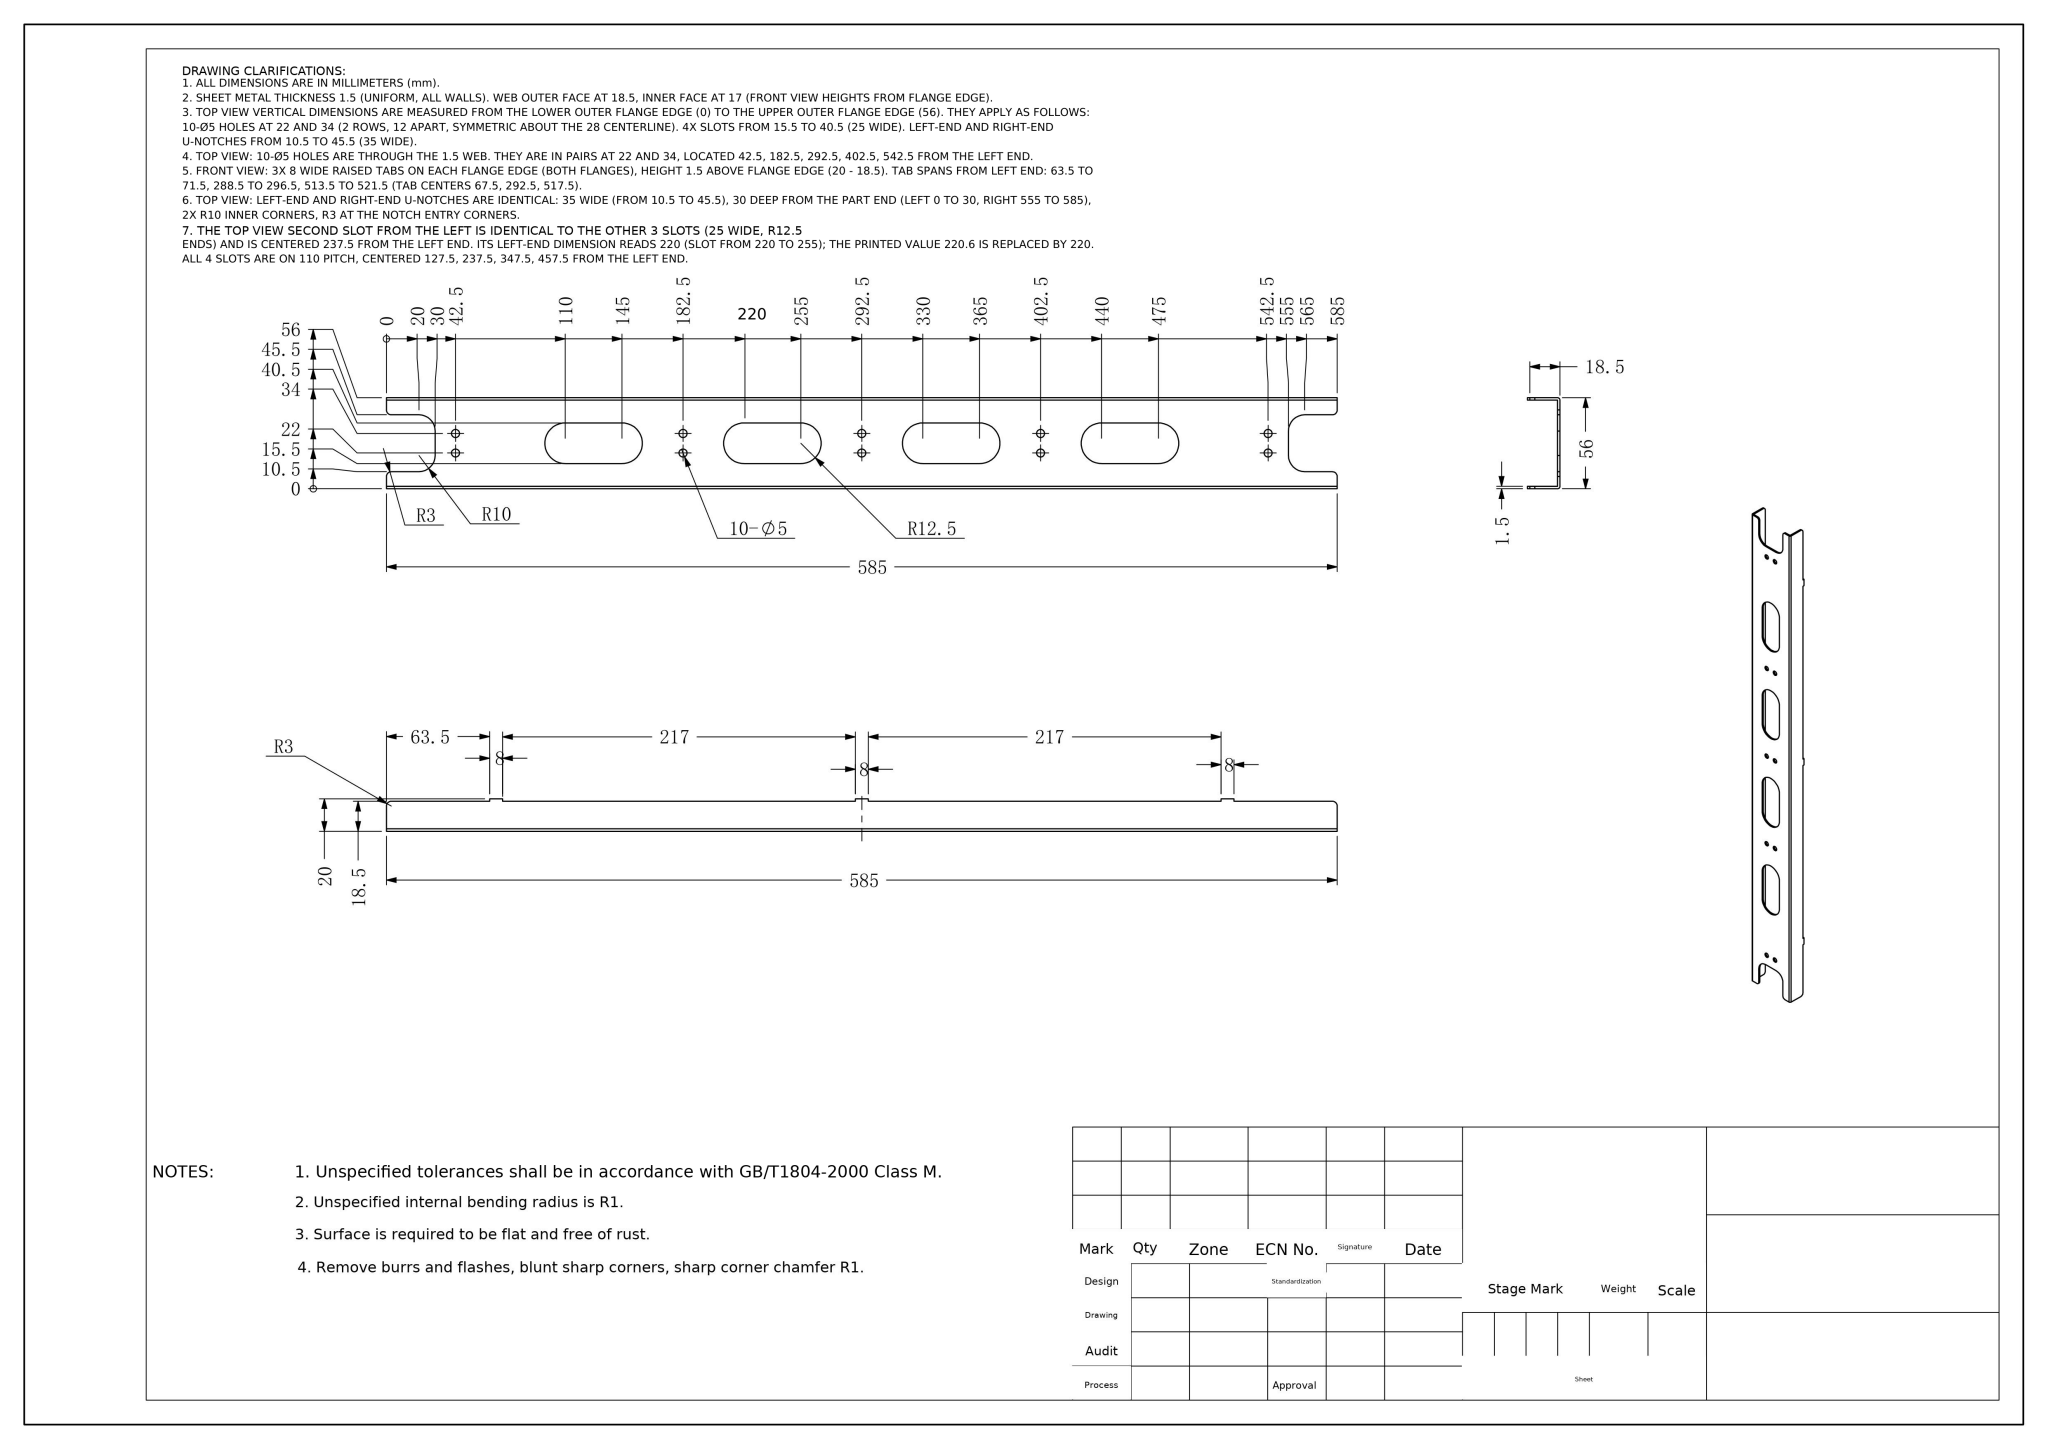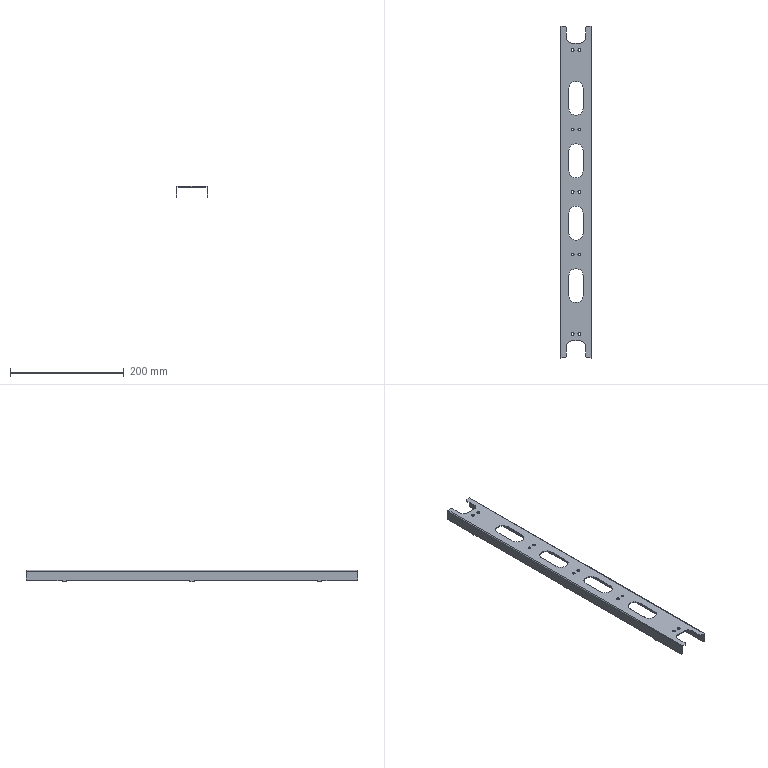Part | NX | mm | 1 solid | 110 faces | box 56 x 585 x 20 mm | volume 66976 mm3 | cylinder 60 | plane 50 | commonest cylinder face diameters 25.028 x24 5 x20 6 x8 20 x4 0.004 x2 3.004 x2